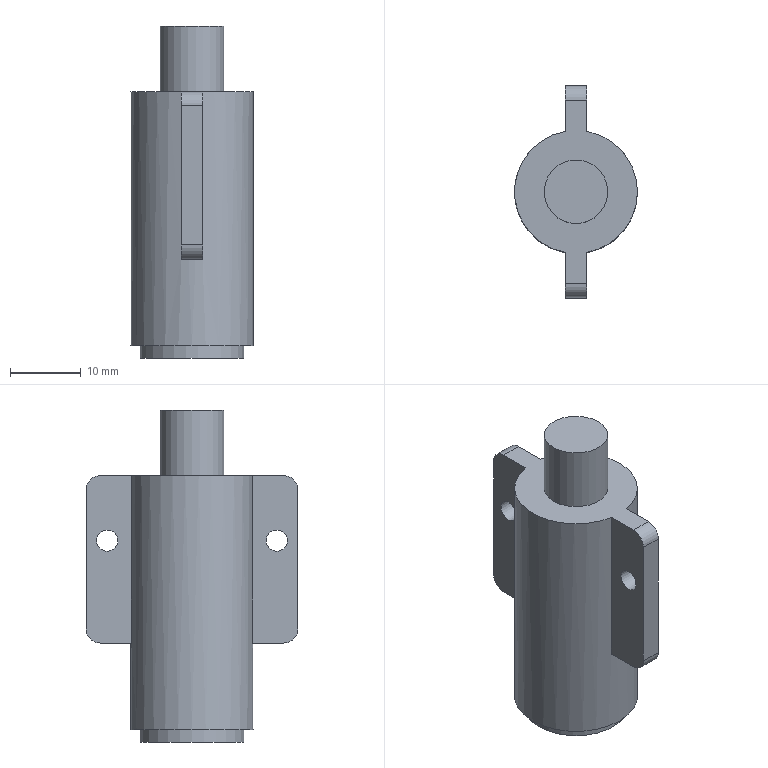Component | NX | SAFETY_BOLT | 1 solid | 21 faces | volume 10290 mm3 | plane 12 | cylinder 9 | commonest cylinder face diameters 4 x4 3 x2 17.4 x1 14.7 x1 9 x1